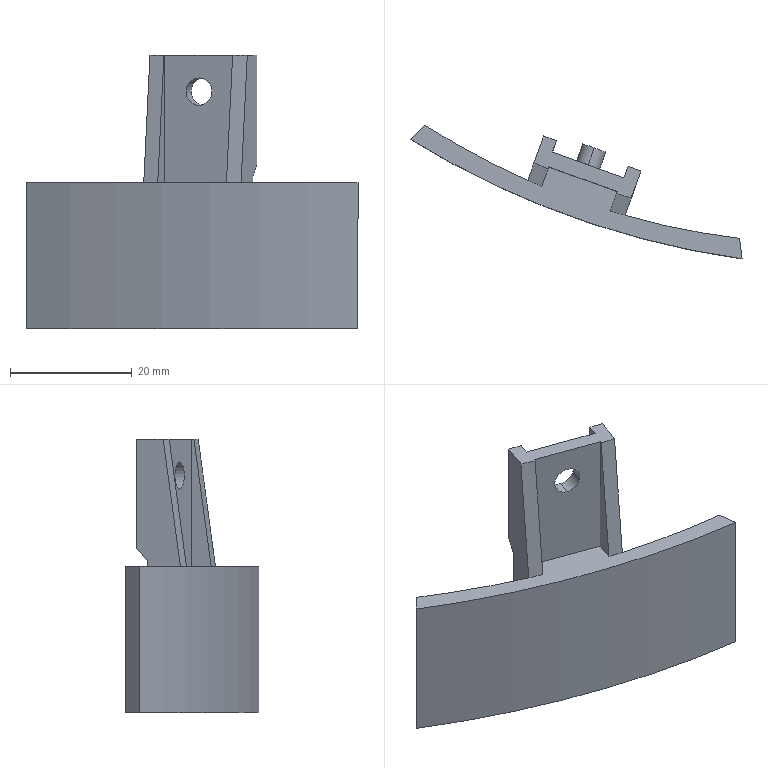Component | SolidWorks | CLS-MechanismIndicatorPlate-1 | 1 solid | 32 faces | box 54.57 x 21.97 x 45 mm | volume 6378 mm3 | plane 23 | cylinder 7 | cone 2 | commonest cylinder face diameters 4 x2 4.5 x2 247.05 x2 283.333 x1
STEP:
#1=CARTESIAN_POINT('',(1.558,-2.417,-0.8662));
#2=VERTEX_POINT('',#1);
#3=CARTESIAN_POINT('',(1.558,-2.417,-0.7087));
#4=VERTEX_POINT('',#3);
#5=CARTESIAN_POINT('',(1.558,-2.417,-0.7874));
#6=DIRECTION('',(0.3389,0.9408,-0.));
#7=DIRECTION('',(0.,-0.,-1.));
#8=AXIS2_PLACEMENT_3D('',#5,#6,#7);
#9=CIRCLE('',#8,0.07874);
#10=EDGE_CURVE('',#2,#4,#9,.T.);
#11=ORIENTED_EDGE('',*,*,#10,.F.);
#12=CARTESIAN_POINT('',(1.518,-2.528,-0.8662));
#13=VERTEX_POINT('',#12);
#14=CARTESIAN_POINT('',(1.558,-2.417,-0.8662));
#15=DIRECTION('',(-0.3389,-0.9408,0.));
#16=VECTOR('',#15,39.37);
#17=LINE('',#14,#16);
#18=EDGE_CURVE('',#2,#13,#17,.T.);
#19=ORIENTED_EDGE('',*,*,#18,.T.);
#20=CARTESIAN_POINT('',(1.518,-2.528,-0.7087));
#21=VERTEX_POINT('',#20);
#22=CARTESIAN_POINT('',(1.518,-2.528,-0.7874));
#23=DIRECTION('',(0.3389,0.9408,-0.));
#24=DIRECTION('',(0.,0.,-1.));
#25=AXIS2_PLACEMENT_3D('',#22,#23,#24);
#26=CIRCLE('',#25,0.07874);
#27=EDGE_CURVE('',#13,#21,#26,.T.);
#28=ORIENTED_EDGE('',*,*,#27,.T.);
#29=CARTESIAN_POINT('',(1.558,-2.417,-0.7087));
#30=DIRECTION('',(-0.3389,-0.9408,0.));
#31=VECTOR('',#30,39.37);
#32=LINE('',#29,#31);
#33=EDGE_CURVE('',#4,#21,#32,.T.);
#34=ORIENTED_EDGE('',*,*,#33,.F.);
#35=EDGE_LOOP('',(#11,#19,#28,#34));
#36=FACE_OUTER_BOUND('',#35,.T.);
#37=CARTESIAN_POINT('',(1.558,-2.417,-0.7874));
#38=DIRECTION('',(-0.3389,-0.9408,0.));
#39=DIRECTION('',(0.,0.,1.));
#40=AXIS2_PLACEMENT_3D('',#37,#38,#39);
#41=CYLINDRICAL_SURFACE('',#40,0.07874);
#42=ADVANCED_FACE('',(#36),#41,.T.);
#43=CARTESIAN_POINT('',(1.485,-2.62,-0.3051));
#44=VERTEX_POINT('',#43);
#45=CARTESIAN_POINT('',(1.485,-2.62,-0.4823));
#46=VERTEX_POINT('',#45);
#47=CARTESIAN_POINT('',(1.485,-2.62,-0.3937));
#48=DIRECTION('',(0.3389,0.9408,-0.));
#49=DIRECTION('',(-0.9408,0.3389,0.));
#50=AXIS2_PLACEMENT_3D('',#47,#48,#49);
#51=CIRCLE('',#50,0.08858);
#52=EDGE_CURVE('',#44,#46,#51,.T.);
#53=ORIENTED_EDGE('',*,*,#52,.F.);
#54=CARTESIAN_POINT('',(1.518,-2.528,-0.3051));
#55=VERTEX_POINT('',#54);
#56=CARTESIAN_POINT('',(1.425,-2.787,-0.3051));
#57=DIRECTION('',(0.3389,0.9408,-0.));
#58=VECTOR('',#57,39.37);
#59=LINE('',#56,#58);
#60=EDGE_CURVE('',#44,#55,#59,.T.);
#61=ORIENTED_EDGE('',*,*,#60,.T.);
#62=CARTESIAN_POINT('',(1.518,-2.528,-0.4823));
#63=VERTEX_POINT('',#62);
#64=CARTESIAN_POINT('',(1.518,-2.528,-0.3937));
#65=DIRECTION('',(0.3389,0.9408,-0.));
#66=DIRECTION('',(0.,-0.,-1.));
#67=AXIS2_PLACEMENT_3D('',#64,#65,#66);
#68=CIRCLE('',#67,0.08858);
#69=EDGE_CURVE('',#55,#63,#68,.T.);
#70=ORIENTED_EDGE('',*,*,#69,.T.);
#71=CARTESIAN_POINT('',(1.425,-2.787,-0.4823));
#72=DIRECTION('',(0.3389,0.9408,-0.));
#73=VECTOR('',#72,39.37);
#74=LINE('',#71,#73);
#75=EDGE_CURVE('',#46,#63,#74,.T.);
#76=ORIENTED_EDGE('',*,*,#75,.F.);
#77=EDGE_LOOP('',(#53,#61,#70,#76));
#78=FACE_OUTER_BOUND('',#77,.T.);
#79=CARTESIAN_POINT('',(1.425,-2.787,-0.3937));
#80=DIRECTION('',(0.3389,0.9408,-0.));
#81=DIRECTION('',(0.,-0.,-1.));
#82=AXIS2_PLACEMENT_3D('',#79,#80,#81);
#83=CYLINDRICAL_SURFACE('',#82,0.08858);
#84=ADVANCED_FACE('',(#78),#83,.F.);
#85=CARTESIAN_POINT('',(1.287,-2.444,-0.9449));
#86=VERTEX_POINT('',#85);
#87=CARTESIAN_POINT('',(1.203,-2.414,-0.9449));
#88=VERTEX_POINT('',#87);
#89=CARTESIAN_POINT('',(1.287,-2.444,-0.9449));
#90=DIRECTION('',(-0.9408,0.3389,0.));
#91=VECTOR('',#90,39.37);
#92=LINE('',#89,#91);
#93=EDGE_CURVE('',#86,#88,#92,.T.);
#94=ORIENTED_EDGE('',*,*,#93,.F.);
#95=CARTESIAN_POINT('',(1.287,-2.444,-0.1575));
#96=VERTEX_POINT('',#95);
#97=CARTESIAN_POINT('',(1.287,-2.444,-0.1575));
#98=DIRECTION('',(-0.,-0.,-1.));
#99=VECTOR('',#98,39.37);
#100=LINE('',#97,#99);
#101=EDGE_CURVE('',#96,#86,#100,.T.);
#102=ORIENTED_EDGE('',*,*,#101,.F.);
#103=CARTESIAN_POINT('',(1.75,-2.611,-0.1575));
#104=VERTEX_POINT('',#103);
#105=CARTESIAN_POINT('',(1.203,-2.414,-0.1575));
#106=DIRECTION('',(-0.9408,0.3389,0.));
#107=VECTOR('',#106,39.37);
#108=LINE('',#105,#107);
#109=EDGE_CURVE('',#104,#96,#108,.T.);
#110=ORIENTED_EDGE('',*,*,#109,.F.);
#111=CARTESIAN_POINT('',(1.75,-2.611,-0.9449));
#112=VERTEX_POINT('',#111);
#113=CARTESIAN_POINT('',(1.75,-2.611,-0.1575));
#114=DIRECTION('',(0.,0.,1.));
#115=VECTOR('',#114,39.37);
#116=LINE('',#113,#115);
#117=EDGE_CURVE('',#112,#104,#116,.T.);
#118=ORIENTED_EDGE('',*,*,#117,.F.);
#119=CARTESIAN_POINT('',(1.833,-2.641,-0.9449));
#120=VERTEX_POINT('',#119);
#121=CARTESIAN_POINT('',(1.833,-2.641,-0.9449));
#122=DIRECTION('',(-0.9408,0.3389,0.));
#123=VECTOR('',#122,39.37);
#124=LINE('',#121,#123);
#125=EDGE_CURVE('',#120,#112,#124,.T.);
#126=ORIENTED_EDGE('',*,*,#125,.F.);
#127=CARTESIAN_POINT('',(1.833,-2.641,-1.929));
#128=VERTEX_POINT('',#127);
#129=CARTESIAN_POINT('',(1.833,-2.641,-0.9843));
#130=DIRECTION('',(-0.,-0.,-1.));
#131=VECTOR('',#130,39.37);
#132=LINE('',#129,#131);
#133=EDGE_CURVE('',#120,#128,#132,.T.);
#134=ORIENTED_EDGE('',*,*,#133,.T.);
#135=CARTESIAN_POINT('',(1.203,-2.414,-1.929));
#136=VERTEX_POINT('',#135);
#137=CARTESIAN_POINT('',(0.4996,-2.161,-1.929));
#138=DIRECTION('',(0.9408,-0.3389,-0.));
#139=VECTOR('',#138,39.37);
#140=LINE('',#137,#139);
#141=EDGE_CURVE('',#136,#128,#140,.T.);
#142=ORIENTED_EDGE('',*,*,#141,.F.);
#143=CARTESIAN_POINT('',(1.203,-2.414,-0.9843));
#144=DIRECTION('',(-0.,-0.,-1.));
#145=VECTOR('',#144,39.37);
#146=LINE('',#143,#145);
#147=EDGE_CURVE('',#88,#136,#146,.T.);
#148=ORIENTED_EDGE('',*,*,#147,.F.);
#149=EDGE_LOOP('',(#94,#102,#110,#118,#126,#134,#142,#148));
#150=FACE_OUTER_BOUND('',#149,.T.);
#151=CARTESIAN_POINT('',(1.314,-2.454,-1.811));
#152=VERTEX_POINT('',#151);
#153=CARTESIAN_POINT('',(1.314,-2.454,-1.095));
#154=VERTEX_POINT('',#153);
#155=CARTESIAN_POINT('',(1.314,-2.454,-1.095));
#156=DIRECTION('',(0.,0.,1.));
#157=VECTOR('',#156,39.37);
#158=LINE('',#155,#157);
#159=EDGE_CURVE('',#152,#154,#158,.T.);
#160=ORIENTED_EDGE('',*,*,#159,.F.);
#161=CARTESIAN_POINT('',(1.722,-2.601,-1.811));
#162=VERTEX_POINT('',#161);
#163=CARTESIAN_POINT('',(1.722,-2.601,-1.811));
#164=DIRECTION('',(-0.9408,0.3389,0.));
#165=VECTOR('',#164,39.37);
#166=LINE('',#163,#165);
#167=EDGE_CURVE('',#162,#152,#166,.T.);
#168=ORIENTED_EDGE('',*,*,#167,.F.);
#169=CARTESIAN_POINT('',(1.722,-2.601,-1.095));
#170=VERTEX_POINT('',#169);
#171=CARTESIAN_POINT('',(1.722,-2.601,-1.095));
#172=DIRECTION('',(-0.,-0.,-1.));
#173=VECTOR('',#172,39.37);
#174=LINE('',#171,#173);
#175=EDGE_CURVE('',#170,#162,#174,.T.);
#176=ORIENTED_EDGE('',*,*,#175,.F.);
#177=CARTESIAN_POINT('',(1.722,-2.601,-1.095));
#178=DIRECTION('',(0.9408,-0.3389,-0.));
#179=VECTOR('',#178,39.37);
#180=LINE('',#177,#179);
#181=EDGE_CURVE('',#154,#170,#180,.T.);
#182=ORIENTED_EDGE('',*,*,#181,.F.);
#183=EDGE_LOOP('',(#160,#168,#176,#182));
#184=FACE_BOUND('',#183,.T.);
#185=CARTESIAN_POINT('',(1.518,-2.528,-0.3937));
#186=DIRECTION('',(0.3389,0.9408,-0.));
#187=DIRECTION('',(0.,-0.,-1.));
#188=AXIS2_PLACEMENT_3D('',#185,#186,#187);
#189=CIRCLE('',#188,0.08858);
#190=EDGE_CURVE('',#63,#55,#189,.T.);
#191=ORIENTED_EDGE('',*,*,#190,.F.);
#192=ORIENTED_EDGE('',*,*,#69,.F.);
#193=EDGE_LOOP('',(#191,#192));
#194=FACE_BOUND('',#193,.T.);
#195=CARTESIAN_POINT('',(1.518,-2.528,-0.7874));
#196=DIRECTION('',(0.3389,0.9408,-0.));
#197=DIRECTION('',(0.,0.,-1.));
#198=AXIS2_PLACEMENT_3D('',#195,#196,#197);
#199=CIRCLE('',#198,0.07874);
#200=EDGE_CURVE('',#21,#13,#199,.T.);
#201=ORIENTED_EDGE('',*,*,#200,.F.);
#202=ORIENTED_EDGE('',*,*,#27,.F.);
#203=EDGE_LOOP('',(#201,#202));
#204=FACE_BOUND('',#203,.T.);
#205=CARTESIAN_POINT('',(0.4996,-2.161,-0.9843));
#206=DIRECTION('',(0.3389,0.9408,-0.));
#207=DIRECTION('',(-0.,-0.,-1.));
#208=AXIS2_PLACEMENT_3D('',#205,#206,#207);
#209=PLANE('',#208);
#210=ADVANCED_FACE('',(#150,#184,#194,#204),#209,.T.);
#211=CARTESIAN_POINT('',(1.258,-2.553,-0.1575));
#212=VERTEX_POINT('',#211);
#213=CARTESIAN_POINT('',(1.218,-2.665,-0.9843));
#214=VERTEX_POINT('',#213);
#215=CARTESIAN_POINT('',(1.258,-2.553,-0.1575));
#216=CARTESIAN_POINT('',(1.246,-2.585,-0.3966));
#217=CARTESIAN_POINT('',(1.235,-2.618,-0.6356));
#218=CARTESIAN_POINT('',(1.223,-2.65,-0.8747));
#219=CARTESIAN_POINT('',(1.221,-2.655,-0.9112));
#220=CARTESIAN_POINT('',(1.22,-2.66,-0.9477));
#221=CARTESIAN_POINT('',(1.218,-2.665,-0.9843));
#222=B_SPLINE_CURVE_WITH_KNOTS('',3,(#215,#216,#217,#218,#219,#220,#221),.UNSPECIFIED.,.F.,.F.,(4,3,4),(0.02067,0.03908,0.04189),.UNSPECIFIED.);
#223=EDGE_CURVE('',#212,#214,#222,.T.);
#224=ORIENTED_EDGE('',*,*,#223,.F.);
#225=CARTESIAN_POINT('',(1.167,-2.514,-0.1575));
#226=VERTEX_POINT('',#225);
#227=CARTESIAN_POINT('',(3.086,1.825,-0.1575));
#228=DIRECTION('',(0.,0.,1.));
#229=DIRECTION('',(0.9408,-0.3389,-0.));
#230=AXIS2_PLACEMENT_3D('',#227,#228,#229);
#231=CIRCLE('',#230,4.745);
#232=EDGE_CURVE('',#226,#212,#231,.T.);
#233=ORIENTED_EDGE('',*,*,#232,.F.);
#234=CARTESIAN_POINT('',(1.127,-2.626,-0.9843));
#235=VERTEX_POINT('',#234);
#236=CARTESIAN_POINT('',(1.127,-2.626,-0.9843));
#237=CARTESIAN_POINT('',(1.141,-2.589,-0.7087));
#238=CARTESIAN_POINT('',(1.154,-2.551,-0.4331));
#239=CARTESIAN_POINT('',(1.167,-2.514,-0.1575));
#240=B_SPLINE_CURVE_WITH_KNOTS('',3,(#236,#237,#238,#239),.UNSPECIFIED.,.F.,.F.,(4,4),(0.,0.02121),.UNSPECIFIED.);
#241=EDGE_CURVE('',#235,#226,#240,.T.);
#242=ORIENTED_EDGE('',*,*,#241,.F.);
#243=CARTESIAN_POINT('',(3.086,1.825,-0.9843));
#244=DIRECTION('',(0.,0.,1.));
#245=DIRECTION('',(0.9408,-0.3389,-0.));
#246=AXIS2_PLACEMENT_3D('',#243,#244,#245);
#247=CIRCLE('',#246,4.863);
#248=EDGE_CURVE('',#235,#214,#247,.T.);
#249=ORIENTED_EDGE('',*,*,#248,.T.);
#250=EDGE_LOOP('',(#224,#233,#242,#249));
#251=FACE_OUTER_BOUND('',#250,.T.);
#252=CARTESIAN_POINT('',(3.086,1.825,-0.1575));
#253=DIRECTION('',(-0.,-0.,-1.));
#254=DIRECTION('',(0.9408,-0.3389,-0.));
#255=AXIS2_PLACEMENT_3D('',#252,#253,#254);
#256=CONICAL_SURFACE('',#255,4.745,0.1419);
#257=ADVANCED_FACE('',(#251),#256,.T.);
#258=CARTESIAN_POINT('',(0.3653,-2.359,-1.929));
#259=VERTEX_POINT('',#258);
#260=CARTESIAN_POINT('',(0.4609,-2.268,-1.929));
#261=VERTEX_POINT('',#260);
#262=CARTESIAN_POINT('',(0.4609,-2.268,-1.929));
#263=DIRECTION('',(0.7239,0.6899,-0.));
#264=VECTOR('',#263,39.37);
#265=LINE('',#262,#264);
#266=EDGE_CURVE('',#259,#261,#265,.T.);
#267=ORIENTED_EDGE('',*,*,#266,.F.);
#268=CARTESIAN_POINT('',(0.3653,-2.359,-0.9843));
#269=VERTEX_POINT('',#268);
#270=CARTESIAN_POINT('',(0.3653,-2.359,-0.9843));
#271=DIRECTION('',(-0.,-0.,-1.));
#272=VECTOR('',#271,39.37);
#273=LINE('',#270,#272);
#274=EDGE_CURVE('',#269,#259,#273,.T.);
#275=ORIENTED_EDGE('',*,*,#274,.F.);
#276=CARTESIAN_POINT('',(0.4609,-2.268,-0.9843));
#277=VERTEX_POINT('',#276);
#278=CARTESIAN_POINT('',(0.4609,-2.268,-0.9843));
#279=DIRECTION('',(0.7239,0.6899,-0.));
#280=VECTOR('',#279,39.37);
#281=LINE('',#278,#280);
#282=EDGE_CURVE('',#269,#277,#281,.T.);
#283=ORIENTED_EDGE('',*,*,#282,.T.);
#284=CARTESIAN_POINT('',(0.4609,-2.268,-0.9843));
#285=DIRECTION('',(-0.,-0.,-1.));
#286=VECTOR('',#285,39.37);
#287=LINE('',#284,#286);
#288=EDGE_CURVE('',#277,#261,#287,.T.);
#289=ORIENTED_EDGE('',*,*,#288,.T.);
#290=EDGE_LOOP('',(#267,#275,#283,#289));
#291=FACE_OUTER_BOUND('',#290,.T.);
#292=CARTESIAN_POINT('',(0.4609,-2.268,-0.9843));
#293=DIRECTION('',(-0.6899,0.7239,-0.));
#294=DIRECTION('',(-0.7239,-0.6899,0.));
#295=AXIS2_PLACEMENT_3D('',#292,#293,#294);
#296=PLANE('',#295);
#297=ADVANCED_FACE('',(#291),#296,.T.);
#298=CARTESIAN_POINT('',(2.514,-3.133,-1.929));
#299=VERTEX_POINT('',#298);
#300=CARTESIAN_POINT('',(3.29,2.39,-1.929));
#301=DIRECTION('',(0.,0.,1.));
#302=DIRECTION('',(-0.9408,0.3389,0.));
#303=AXIS2_PLACEMENT_3D('',#300,#301,#302);
#304=CIRCLE('',#303,5.577);
#305=EDGE_CURVE('',#259,#299,#304,.T.);
#306=ORIENTED_EDGE('',*,*,#305,.T.);
#307=CARTESIAN_POINT('',(2.514,-3.133,-0.9843));
#308=VERTEX_POINT('',#307);
#309=CARTESIAN_POINT('',(2.514,-3.133,-0.9843));
#310=DIRECTION('',(-0.,-0.,-1.));
#311=VECTOR('',#310,39.37);
#312=LINE('',#309,#311);
#313=EDGE_CURVE('',#308,#299,#312,.T.);
#314=ORIENTED_EDGE('',*,*,#313,.F.);
#315=CARTESIAN_POINT('',(3.29,2.39,-0.9843));
#316=DIRECTION('',(0.,0.,1.));
#317=DIRECTION('',(-0.9408,0.3389,0.));
#318=AXIS2_PLACEMENT_3D('',#315,#316,#317);
#319=CIRCLE('',#318,5.577);
#320=EDGE_CURVE('',#269,#308,#319,.T.);
#321=ORIENTED_EDGE('',*,*,#320,.F.);
#322=ORIENTED_EDGE('',*,*,#274,.T.);
#323=EDGE_LOOP('',(#306,#314,#321,#322));
#324=FACE_OUTER_BOUND('',#323,.T.);
#325=CARTESIAN_POINT('',(3.29,2.39,-0.9843));
#326=DIRECTION('',(-0.,-0.,-1.));
#327=DIRECTION('',(0.9408,-0.3389,-0.));
#328=AXIS2_PLACEMENT_3D('',#325,#326,#327);
#329=CYLINDRICAL_SURFACE('',#328,5.577);
#330=ADVANCED_FACE('',(#324),#329,.T.);
#331=CARTESIAN_POINT('',(2.498,-3.002,-1.929));
#332=VERTEX_POINT('',#331);
#333=CARTESIAN_POINT('',(2.384,-2.04,-1.929));
#334=DIRECTION('',(-0.1176,0.9931,-0.));
#335=VECTOR('',#334,39.37);
#336=LINE('',#333,#335);
#337=EDGE_CURVE('',#299,#332,#336,.T.);
#338=ORIENTED_EDGE('',*,*,#337,.T.);
#339=CARTESIAN_POINT('',(2.498,-3.002,-0.9843));
#340=VERTEX_POINT('',#339);
#341=CARTESIAN_POINT('',(2.498,-3.002,-0.9843));
#342=DIRECTION('',(-0.,-0.,-1.));
#343=VECTOR('',#342,39.37);
#344=LINE('',#341,#343);
#345=EDGE_CURVE('',#340,#332,#344,.T.);
#346=ORIENTED_EDGE('',*,*,#345,.F.);
#347=CARTESIAN_POINT('',(2.384,-2.04,-0.9843));
#348=DIRECTION('',(-0.1176,0.9931,-0.));
#349=VECTOR('',#348,39.37);
#350=LINE('',#347,#349);
#351=EDGE_CURVE('',#308,#340,#350,.T.);
#352=ORIENTED_EDGE('',*,*,#351,.F.);
#353=ORIENTED_EDGE('',*,*,#313,.T.);
#354=EDGE_LOOP('',(#338,#346,#352,#353));
#355=FACE_OUTER_BOUND('',#354,.T.);
#356=CARTESIAN_POINT('',(2.384,-2.04,-0.9843));
#357=DIRECTION('',(-0.9931,-0.1176,0.));
#358=DIRECTION('',(0.1176,-0.9931,0.));
#359=AXIS2_PLACEMENT_3D('',#356,#357,#358);
#360=PLANE('',#359);
#361=ADVANCED_FACE('',(#355),#360,.F.);
#362=CARTESIAN_POINT('',(1.757,-2.853,-1.929));
#363=VERTEX_POINT('',#362);
#364=CARTESIAN_POINT('',(3.086,1.825,-1.929));
#365=DIRECTION('',(0.,0.,1.));
#366=DIRECTION('',(-0.9408,0.3389,0.));
#367=AXIS2_PLACEMENT_3D('',#364,#365,#366);
#368=CIRCLE('',#367,4.863);
#369=EDGE_CURVE('',#363,#332,#368,.T.);
#370=ORIENTED_EDGE('',*,*,#369,.F.);
#371=CARTESIAN_POINT('',(1.757,-2.853,-0.9843));
#372=VERTEX_POINT('',#371);
#373=CARTESIAN_POINT('',(1.757,-2.853,-0.9843));
#374=DIRECTION('',(-0.,-0.,-1.));
#375=VECTOR('',#374,39.37);
#376=LINE('',#373,#375);
#377=EDGE_CURVE('',#372,#363,#376,.T.);
#378=ORIENTED_EDGE('',*,*,#377,.F.);
#379=CARTESIAN_POINT('',(3.086,1.825,-0.9843));
#380=DIRECTION('',(0.,0.,1.));
#381=DIRECTION('',(-0.9408,0.3389,0.));
#382=AXIS2_PLACEMENT_3D('',#379,#380,#381);
#383=CIRCLE('',#382,4.863);
#384=EDGE_CURVE('',#372,#340,#383,.T.);
#385=ORIENTED_EDGE('',*,*,#384,.T.);
#386=ORIENTED_EDGE('',*,*,#345,.T.);
#387=EDGE_LOOP('',(#370,#378,#385,#386));
#388=FACE_OUTER_BOUND('',#387,.T.);
#389=CARTESIAN_POINT('',(3.086,1.825,-0.9843));
#390=DIRECTION('',(-0.,-0.,-1.));
#391=DIRECTION('',(0.9408,-0.3389,-0.));
#392=AXIS2_PLACEMENT_3D('',#389,#390,#391);
#393=CYLINDRICAL_SURFACE('',#392,4.863);
#394=ADVANCED_FACE('',(#388),#393,.F.);
#395=CARTESIAN_POINT('',(1.797,-2.741,-0.1575));
#396=VERTEX_POINT('',#395);
#397=CARTESIAN_POINT('',(1.86,-2.567,-0.1575));
#398=VERTEX_POINT('',#397);
#399=CARTESIAN_POINT('',(1.833,-2.641,-0.1575));
#400=DIRECTION('',(0.3389,0.9408,-0.));
#401=VECTOR('',#400,39.37);
#402=LINE('',#399,#401);
#403=EDGE_CURVE('',#396,#398,#402,.T.);
#404=ORIENTED_EDGE('',*,*,#403,.F.);
#405=CARTESIAN_POINT('',(1.797,-2.741,-0.1575));
#406=CARTESIAN_POINT('',(1.784,-2.778,-0.4331));
#407=CARTESIAN_POINT('',(1.77,-2.815,-0.7087));
#408=CARTESIAN_POINT('',(1.757,-2.853,-0.9843));
#409=B_SPLINE_CURVE_WITH_KNOTS('',3,(#405,#406,#407,#408),.UNSPECIFIED.,.F.,.F.,(4,4),(0.,0.02121),.UNSPECIFIED.);
#410=EDGE_CURVE('',#396,#372,#409,.T.);
#411=ORIENTED_EDGE('',*,*,#410,.T.);
#412=ORIENTED_EDGE('',*,*,#377,.T.);
#413=CARTESIAN_POINT('',(1.794,-2.749,-1.929));
#414=DIRECTION('',(0.3389,0.9408,-0.));
#415=VECTOR('',#414,39.37);
#416=LINE('',#413,#415);
#417=EDGE_CURVE('',#363,#128,#416,.T.);
#418=ORIENTED_EDGE('',*,*,#417,.T.);
#419=ORIENTED_EDGE('',*,*,#133,.F.);
#420=CARTESIAN_POINT('',(1.86,-2.567,-0.8662));
#421=VERTEX_POINT('',#420);
#422=CARTESIAN_POINT('',(1.86,-2.567,-0.8662));
#423=DIRECTION('',(0.2396,0.6653,0.7071));
#424=VECTOR('',#423,39.37);
#425=LINE('',#422,#424);
#426=EDGE_CURVE('',#120,#421,#425,.T.);
#427=ORIENTED_EDGE('',*,*,#426,.T.);
#428=CARTESIAN_POINT('',(1.86,-2.567,-0.1575));
#429=DIRECTION('',(-0.,-0.,-1.));
#430=VECTOR('',#429,39.37);
#431=LINE('',#428,#430);
#432=EDGE_CURVE('',#398,#421,#431,.T.);
#433=ORIENTED_EDGE('',*,*,#432,.F.);
#434=EDGE_LOOP('',(#404,#411,#412,#418,#419,#427,#433));
#435=FACE_OUTER_BOUND('',#434,.T.);
#436=CARTESIAN_POINT('',(1.794,-2.749,-0.9843));
#437=DIRECTION('',(-0.9408,0.3389,0.));
#438=DIRECTION('',(-0.,-0.,-1.));
#439=AXIS2_PLACEMENT_3D('',#436,#437,#438);
#440=PLANE('',#439);
#441=ADVANCED_FACE('',(#435),#440,.F.);
#442=CARTESIAN_POINT('',(1.127,-2.626,-1.929));
#443=VERTEX_POINT('',#442);
#444=CARTESIAN_POINT('',(1.127,-2.626,-0.9843));
#445=DIRECTION('',(-0.,-0.,-1.));
#446=VECTOR('',#445,39.37);
#447=LINE('',#444,#446);
#448=EDGE_CURVE('',#235,#443,#447,.T.);
#449=ORIENTED_EDGE('',*,*,#448,.F.);
#450=ORIENTED_EDGE('',*,*,#241,.T.);
#451=CARTESIAN_POINT('',(1.23,-2.34,-0.1575));
#452=VERTEX_POINT('',#451);
#453=CARTESIAN_POINT('',(1.203,-2.414,-0.1575));
#454=DIRECTION('',(-0.3389,-0.9408,0.));
#455=VECTOR('',#454,39.37);
#456=LINE('',#453,#455);
#457=EDGE_CURVE('',#452,#226,#456,.T.);
#458=ORIENTED_EDGE('',*,*,#457,.F.);
#459=CARTESIAN_POINT('',(1.23,-2.34,-0.8662));
#460=VERTEX_POINT('',#459);
#461=CARTESIAN_POINT('',(1.23,-2.34,-0.1575));
#462=DIRECTION('',(0.,0.,1.));
#463=VECTOR('',#462,39.37);
#464=LINE('',#461,#463);
#465=EDGE_CURVE('',#460,#452,#464,.T.);
#466=ORIENTED_EDGE('',*,*,#465,.F.);
#467=CARTESIAN_POINT('',(1.177,-2.487,-1.022));
#468=DIRECTION('',(-0.2396,-0.6653,-0.7071));
#469=VECTOR('',#468,39.37);
#470=LINE('',#467,#469);
#471=EDGE_CURVE('',#460,#88,#470,.T.);
#472=ORIENTED_EDGE('',*,*,#471,.T.);
#473=ORIENTED_EDGE('',*,*,#147,.T.);
#474=CARTESIAN_POINT('',(1.165,-2.522,-1.929));
#475=DIRECTION('',(0.3389,0.9408,-0.));
#476=VECTOR('',#475,39.37);
#477=LINE('',#474,#476);
#478=EDGE_CURVE('',#443,#136,#477,.T.);
#479=ORIENTED_EDGE('',*,*,#478,.F.);
#480=EDGE_LOOP('',(#449,#450,#458,#466,#472,#473,#479));
#481=FACE_OUTER_BOUND('',#480,.T.);
#482=CARTESIAN_POINT('',(1.165,-2.522,-0.9843));
#483=DIRECTION('',(-0.9408,0.3389,0.));
#484=DIRECTION('',(-0.,-0.,-1.));
#485=AXIS2_PLACEMENT_3D('',#482,#483,#484);
#486=PLANE('',#485);
#487=ADVANCED_FACE('',(#481),#486,.T.);
#488=CARTESIAN_POINT('',(3.086,1.825,-1.929));
#489=DIRECTION('',(0.,0.,1.));
#490=DIRECTION('',(-0.9408,0.3389,0.));
#491=AXIS2_PLACEMENT_3D('',#488,#489,#490);
#492=CIRCLE('',#491,4.863);
#493=EDGE_CURVE('',#261,#443,#492,.T.);
#494=ORIENTED_EDGE('',*,*,#493,.F.);
#495=ORIENTED_EDGE('',*,*,#288,.F.);
#496=CARTESIAN_POINT('',(3.086,1.825,-0.9843));
#497=DIRECTION('',(0.,0.,1.));
#498=DIRECTION('',(-0.9408,0.3389,0.));
#499=AXIS2_PLACEMENT_3D('',#496,#497,#498);
#500=CIRCLE('',#499,4.863);
#501=EDGE_CURVE('',#277,#235,#500,.T.);
#502=ORIENTED_EDGE('',*,*,#501,.T.);
#503=ORIENTED_EDGE('',*,*,#448,.T.);
#504=EDGE_LOOP('',(#494,#495,#502,#503));
#505=FACE_OUTER_BOUND('',#504,.T.);
#506=CARTESIAN_POINT('',(3.086,1.825,-0.9843));
#507=DIRECTION('',(-0.,-0.,-1.));
#508=DIRECTION('',(0.9408,-0.3389,-0.));
#509=AXIS2_PLACEMENT_3D('',#506,#507,#508);
#510=CYLINDRICAL_SURFACE('',#509,4.863);
#511=ADVANCED_FACE('',(#505),#510,.F.);
#512=CARTESIAN_POINT('',(1.662,-2.825,-0.9843));
#513=VERTEX_POINT('',#512);
#514=CARTESIAN_POINT('',(3.086,1.825,-0.9843));
#515=DIRECTION('',(0.,0.,1.));
#516=DIRECTION('',(0.9408,-0.3389,-0.));
#517=AXIS2_PLACEMENT_3D('',#514,#515,#516);
#518=CIRCLE('',#517,4.863);
#519=EDGE_CURVE('',#513,#372,#518,.T.);
#520=ORIENTED_EDGE('',*,*,#519,.F.);
#521=CARTESIAN_POINT('',(1.707,-2.7,-0.9843));
#522=VERTEX_POINT('',#521);
#523=CARTESIAN_POINT('',(1.707,-2.7,-0.9843));
#524=DIRECTION('',(0.3389,0.9408,-0.));
#525=VECTOR('',#524,39.37);
#526=LINE('',#523,#525);
#527=EDGE_CURVE('',#513,#522,#526,.T.);
#528=ORIENTED_EDGE('',*,*,#527,.T.);
#529=CARTESIAN_POINT('',(1.263,-2.54,-0.9843));
#530=VERTEX_POINT('',#529);
#531=CARTESIAN_POINT('',(1.263,-2.54,-0.9843));
#532=DIRECTION('',(-0.9408,0.3389,0.));
#533=VECTOR('',#532,39.37);
#534=LINE('',#531,#533);
#535=EDGE_CURVE('',#522,#530,#534,.T.);
#536=ORIENTED_EDGE('',*,*,#535,.T.);
#537=CARTESIAN_POINT('',(1.263,-2.54,-0.9843));
#538=DIRECTION('',(-0.3389,-0.9408,0.));
#539=VECTOR('',#538,39.37);
#540=LINE('',#537,#539);
#541=EDGE_CURVE('',#530,#214,#540,.T.);
#542=ORIENTED_EDGE('',*,*,#541,.T.);
#543=ORIENTED_EDGE('',*,*,#248,.F.);
#544=ORIENTED_EDGE('',*,*,#501,.F.);
#545=ORIENTED_EDGE('',*,*,#282,.F.);
#546=ORIENTED_EDGE('',*,*,#320,.T.);
#547=ORIENTED_EDGE('',*,*,#351,.T.);
#548=ORIENTED_EDGE('',*,*,#384,.F.);
#549=EDGE_LOOP('',(#520,#528,#536,#542,#543,#544,#545,#546,#547,#548));
#550=FACE_OUTER_BOUND('',#549,.T.);
#551=CARTESIAN_POINT('',(0.4609,-2.268,-0.9843));
#552=DIRECTION('',(0.,0.,1.));
#553=DIRECTION('',(-0.9408,0.3389,0.));
#554=AXIS2_PLACEMENT_3D('',#551,#552,#553);
#555=PLANE('',#554);
#556=ADVANCED_FACE('',(#550),#555,.T.);
#557=ORIENTED_EDGE('',*,*,#266,.T.);
#558=ORIENTED_EDGE('',*,*,#493,.T.);
#559=ORIENTED_EDGE('',*,*,#478,.T.);
#560=ORIENTED_EDGE('',*,*,#141,.T.);
#561=ORIENTED_EDGE('',*,*,#417,.F.);
#562=ORIENTED_EDGE('',*,*,#369,.T.);
#563=ORIENTED_EDGE('',*,*,#337,.F.);
#564=ORIENTED_EDGE('',*,*,#305,.F.);
#565=EDGE_LOOP('',(#557,#558,#559,#560,#561,#562,#563,#564));
#566=FACE_OUTER_BOUND('',#565,.T.);
#567=CARTESIAN_POINT('',(0.4609,-2.268,-1.929));
#568=DIRECTION('',(0.,0.,1.));
#569=DIRECTION('',(-0.9408,0.3389,0.));
#570=AXIS2_PLACEMENT_3D('',#567,#568,#569);
#571=PLANE('',#570);
#572=ADVANCED_FACE('',(#566),#571,.F.);
#573=ORIENTED_EDGE('',*,*,#232,.T.);
#574=CARTESIAN_POINT('',(1.263,-2.54,-0.1575));
#575=VERTEX_POINT('',#574);
#576=CARTESIAN_POINT('',(1.263,-2.54,-0.1575));
#577=DIRECTION('',(-0.3389,-0.9408,0.));
#578=VECTOR('',#577,39.37);
#579=LINE('',#576,#578);
#580=EDGE_CURVE('',#575,#212,#579,.T.);
#581=ORIENTED_EDGE('',*,*,#580,.F.);
#582=CARTESIAN_POINT('',(1.707,-2.7,-0.1575));
#583=VERTEX_POINT('',#582);
#584=CARTESIAN_POINT('',(1.263,-2.54,-0.1575));
#585=DIRECTION('',(-0.9408,0.3389,0.));
#586=VECTOR('',#585,39.37);
#587=LINE('',#584,#586);
#588=EDGE_CURVE('',#583,#575,#587,.T.);
#589=ORIENTED_EDGE('',*,*,#588,.F.);
#590=CARTESIAN_POINT('',(1.702,-2.713,-0.1575));
#591=VERTEX_POINT('',#590);
#592=CARTESIAN_POINT('',(1.707,-2.7,-0.1575));
#593=DIRECTION('',(0.3389,0.9408,-0.));
#594=VECTOR('',#593,39.37);
#595=LINE('',#592,#594);
#596=EDGE_CURVE('',#591,#583,#595,.T.);
#597=ORIENTED_EDGE('',*,*,#596,.F.);
#598=CARTESIAN_POINT('',(3.086,1.825,-0.1575));
#599=DIRECTION('',(0.,0.,1.));
#600=DIRECTION('',(0.9408,-0.3389,-0.));
#601=AXIS2_PLACEMENT_3D('',#598,#599,#600);
#602=CIRCLE('',#601,4.745);
#603=EDGE_CURVE('',#591,#396,#602,.T.);
#604=ORIENTED_EDGE('',*,*,#603,.T.);
#605=ORIENTED_EDGE('',*,*,#403,.T.);
#606=CARTESIAN_POINT('',(1.776,-2.537,-0.1575));
#607=VERTEX_POINT('',#606);
#608=CARTESIAN_POINT('',(1.86,-2.567,-0.1575));
#609=DIRECTION('',(0.9408,-0.3389,-0.));
#610=VECTOR('',#609,39.37);
#611=LINE('',#608,#610);
#612=EDGE_CURVE('',#607,#398,#611,.T.);
#613=ORIENTED_EDGE('',*,*,#612,.F.);
#614=CARTESIAN_POINT('',(1.776,-2.537,-0.1575));
#615=DIRECTION('',(-0.3389,-0.9408,0.));
#616=VECTOR('',#615,39.37);
#617=LINE('',#614,#616);
#618=EDGE_CURVE('',#607,#104,#617,.T.);
#619=ORIENTED_EDGE('',*,*,#618,.T.);
#620=ORIENTED_EDGE('',*,*,#109,.T.);
#621=CARTESIAN_POINT('',(1.313,-2.37,-0.1575));
#622=VERTEX_POINT('',#621);
#623=CARTESIAN_POINT('',(1.313,-2.37,-0.1575));
#624=DIRECTION('',(-0.3389,-0.9408,0.));
#625=VECTOR('',#624,39.37);
#626=LINE('',#623,#625);
#627=EDGE_CURVE('',#622,#96,#626,.T.);
#628=ORIENTED_EDGE('',*,*,#627,.F.);
#629=CARTESIAN_POINT('',(1.313,-2.37,-0.1575));
#630=DIRECTION('',(0.9408,-0.3389,-0.));
#631=VECTOR('',#630,39.37);
#632=LINE('',#629,#631);
#633=EDGE_CURVE('',#452,#622,#632,.T.);
#634=ORIENTED_EDGE('',*,*,#633,.F.);
#635=ORIENTED_EDGE('',*,*,#457,.T.);
#636=EDGE_LOOP('',(#573,#581,#589,#597,#604,#605,#613,#619,#620,#628,#634,#635));
#637=FACE_OUTER_BOUND('',#636,.T.);
#638=CARTESIAN_POINT('',(3.086,1.825,-0.1575));
#639=DIRECTION('',(-0.,-0.,-1.));
#640=DIRECTION('',(0.9408,-0.3389,-0.));
#641=AXIS2_PLACEMENT_3D('',#638,#639,#640);
#642=PLANE('',#641);
#643=ADVANCED_FACE('',(#637),#642,.F.);
#644=CARTESIAN_POINT('',(1.776,-2.537,-0.8662));
#645=VERTEX_POINT('',#644);
#646=CARTESIAN_POINT('',(1.776,-2.537,-0.1575));
#647=DIRECTION('',(0.,0.,1.));
#648=VECTOR('',#647,39.37);
#649=LINE('',#646,#648);
#650=EDGE_CURVE('',#645,#607,#649,.T.);
#651=ORIENTED_EDGE('',*,*,#650,.F.);
#652=CARTESIAN_POINT('',(1.776,-2.537,-0.8662));
#653=DIRECTION('',(-0.2396,-0.6653,-0.7071));
#654=VECTOR('',#653,39.37);
#655=LINE('',#652,#654);
#656=EDGE_CURVE('',#645,#112,#655,.T.);
#657=ORIENTED_EDGE('',*,*,#656,.T.);
#658=ORIENTED_EDGE('',*,*,#117,.T.);
#659=ORIENTED_EDGE('',*,*,#618,.F.);
#660=EDGE_LOOP('',(#651,#657,#658,#659));
#661=FACE_OUTER_BOUND('',#660,.T.);
#662=CARTESIAN_POINT('',(1.776,-2.537,-0.1575));
#663=DIRECTION('',(0.9408,-0.3389,-0.));
#664=DIRECTION('',(0.,0.,1.));
#665=AXIS2_PLACEMENT_3D('',#662,#663,#664);
#666=PLANE('',#665);
#667=ADVANCED_FACE('',(#661),#666,.F.);
#668=ORIENTED_EDGE('',*,*,#432,.T.);
#669=CARTESIAN_POINT('',(1.776,-2.537,-0.8662));
#670=DIRECTION('',(-0.9408,0.3389,0.));
#671=VECTOR('',#670,39.37);
#672=LINE('',#669,#671);
#673=EDGE_CURVE('',#421,#645,#672,.T.);
#674=ORIENTED_EDGE('',*,*,#673,.T.);
#675=ORIENTED_EDGE('',*,*,#650,.T.);
#676=ORIENTED_EDGE('',*,*,#612,.T.);
#677=EDGE_LOOP('',(#668,#674,#675,#676));
#678=FACE_OUTER_BOUND('',#677,.T.);
#679=CARTESIAN_POINT('',(1.776,-2.537,-0.1575));
#680=DIRECTION('',(-0.3389,-0.9408,0.));
#681=DIRECTION('',(0.,0.,1.));
#682=AXIS2_PLACEMENT_3D('',#679,#680,#681);
#683=PLANE('',#682);
#684=ADVANCED_FACE('',(#678),#683,.F.);
#685=ORIENTED_EDGE('',*,*,#101,.T.);
#686=CARTESIAN_POINT('',(1.313,-2.37,-0.8662));
#687=VERTEX_POINT('',#686);
#688=CARTESIAN_POINT('',(1.313,-2.37,-0.8662));
#689=DIRECTION('',(0.2396,0.6653,0.7071));
#690=VECTOR('',#689,39.37);
#691=LINE('',#688,#690);
#692=EDGE_CURVE('',#86,#687,#691,.T.);
#693=ORIENTED_EDGE('',*,*,#692,.T.);
#694=CARTESIAN_POINT('',(1.313,-2.37,-0.1575));
#695=DIRECTION('',(-0.,-0.,-1.));
#696=VECTOR('',#695,39.37);
#697=LINE('',#694,#696);
#698=EDGE_CURVE('',#622,#687,#697,.T.);
#699=ORIENTED_EDGE('',*,*,#698,.F.);
#700=ORIENTED_EDGE('',*,*,#627,.T.);
#701=EDGE_LOOP('',(#685,#693,#699,#700));
#702=FACE_OUTER_BOUND('',#701,.T.);
#703=CARTESIAN_POINT('',(1.313,-2.37,-0.1575));
#704=DIRECTION('',(-0.9408,0.3389,0.));
#705=DIRECTION('',(-0.,-0.,-1.));
#706=AXIS2_PLACEMENT_3D('',#703,#704,#705);
#707=PLANE('',#706);
#708=ADVANCED_FACE('',(#702),#707,.F.);
#709=ORIENTED_EDGE('',*,*,#698,.T.);
#710=CARTESIAN_POINT('',(1.23,-2.34,-0.8662));
#711=DIRECTION('',(-0.9408,0.3389,0.));
#712=VECTOR('',#711,39.37);
#713=LINE('',#710,#712);
#714=EDGE_CURVE('',#687,#460,#713,.T.);
#715=ORIENTED_EDGE('',*,*,#714,.T.);
#716=ORIENTED_EDGE('',*,*,#465,.T.);
#717=ORIENTED_EDGE('',*,*,#633,.T.);
#718=EDGE_LOOP('',(#709,#715,#716,#717));
#719=FACE_OUTER_BOUND('',#718,.T.);
#720=CARTESIAN_POINT('',(1.313,-2.37,-0.9449));
#721=DIRECTION('',(0.3389,0.9408,-0.));
#722=DIRECTION('',(-0.,-0.,-1.));
#723=AXIS2_PLACEMENT_3D('',#720,#721,#722);
#724=PLANE('',#723);
#725=ADVANCED_FACE('',(#719),#724,.T.);
#726=ORIENTED_EDGE('',*,*,#426,.F.);
#727=ORIENTED_EDGE('',*,*,#125,.T.);
#728=ORIENTED_EDGE('',*,*,#656,.F.);
#729=ORIENTED_EDGE('',*,*,#673,.F.);
#730=EDGE_LOOP('',(#726,#727,#728,#729));
#731=FACE_OUTER_BOUND('',#730,.T.);
#732=CARTESIAN_POINT('',(1.776,-2.537,-0.8662));
#733=DIRECTION('',(-0.2396,-0.6653,0.7071));
#734=DIRECTION('',(0.2396,0.6653,0.7071));
#735=AXIS2_PLACEMENT_3D('',#732,#733,#734);
#736=PLANE('',#735);
#737=ADVANCED_FACE('',(#731),#736,.F.);
#738=ORIENTED_EDGE('',*,*,#692,.F.);
#739=ORIENTED_EDGE('',*,*,#93,.T.);
#740=ORIENTED_EDGE('',*,*,#471,.F.);
#741=ORIENTED_EDGE('',*,*,#714,.F.);
#742=EDGE_LOOP('',(#738,#739,#740,#741));
#743=FACE_OUTER_BOUND('',#742,.T.);
#744=CARTESIAN_POINT('',(1.313,-2.37,-0.8662));
#745=DIRECTION('',(0.2396,0.6653,-0.7071));
#746=DIRECTION('',(-0.2396,-0.6653,-0.7071));
#747=AXIS2_PLACEMENT_3D('',#744,#745,#746);
#748=PLANE('',#747);
#749=ADVANCED_FACE('',(#743),#748,.T.);
#750=CARTESIAN_POINT('',(1.662,-2.825,-0.9843));
#751=CARTESIAN_POINT('',(1.664,-2.82,-0.9477));
#752=CARTESIAN_POINT('',(1.666,-2.815,-0.9112));
#753=CARTESIAN_POINT('',(1.668,-2.81,-0.8747));
#754=CARTESIAN_POINT('',(1.679,-2.778,-0.6356));
#755=CARTESIAN_POINT('',(1.691,-2.746,-0.3966));
#756=CARTESIAN_POINT('',(1.702,-2.713,-0.1575));
#757=B_SPLINE_CURVE_WITH_KNOTS('',3,(#750,#751,#752,#753,#754,#755,#756),.UNSPECIFIED.,.F.,.F.,(4,3,4),(0.03626,0.03908,0.05748),.UNSPECIFIED.);
#758=EDGE_CURVE('',#513,#591,#757,.T.);
#759=ORIENTED_EDGE('',*,*,#758,.F.);
#760=ORIENTED_EDGE('',*,*,#519,.T.);
#761=ORIENTED_EDGE('',*,*,#410,.F.);
#762=ORIENTED_EDGE('',*,*,#603,.F.);
#763=EDGE_LOOP('',(#759,#760,#761,#762));
#764=FACE_OUTER_BOUND('',#763,.T.);
#765=CARTESIAN_POINT('',(3.086,1.825,-0.1575));
#766=DIRECTION('',(-0.,-0.,-1.));
#767=DIRECTION('',(0.9408,-0.3389,-0.));
#768=AXIS2_PLACEMENT_3D('',#765,#766,#767);
#769=CONICAL_SURFACE('',#768,4.745,0.1419);
#770=ADVANCED_FACE('',(#764),#769,.T.);
#771=ORIENTED_EDGE('',*,*,#223,.T.);
#772=ORIENTED_EDGE('',*,*,#541,.F.);
#773=CARTESIAN_POINT('',(1.263,-2.54,-0.9843));
#774=DIRECTION('',(0.,0.,1.));
#775=VECTOR('',#774,39.37);
#776=LINE('',#773,#775);
#777=EDGE_CURVE('',#530,#575,#776,.T.);
#778=ORIENTED_EDGE('',*,*,#777,.T.);
#779=ORIENTED_EDGE('',*,*,#580,.T.);
#780=EDGE_LOOP('',(#771,#772,#778,#779));
#781=FACE_OUTER_BOUND('',#780,.T.);
#782=CARTESIAN_POINT('',(1.263,-2.54,-0.9843));
#783=DIRECTION('',(-0.9408,0.3389,0.));
#784=DIRECTION('',(-0.,-0.,-1.));
#785=AXIS2_PLACEMENT_3D('',#782,#783,#784);
#786=PLANE('',#785);
#787=ADVANCED_FACE('',(#781),#786,.F.);
#788=CARTESIAN_POINT('',(1.485,-2.62,-0.3937));
#789=DIRECTION('',(0.3389,0.9408,-0.));
#790=DIRECTION('',(-0.9408,0.3389,0.));
#791=AXIS2_PLACEMENT_3D('',#788,#789,#790);
#792=CIRCLE('',#791,0.08858);
#793=EDGE_CURVE('',#46,#44,#792,.T.);
#794=ORIENTED_EDGE('',*,*,#793,.T.);
#795=ORIENTED_EDGE('',*,*,#52,.T.);
#796=EDGE_LOOP('',(#794,#795));
#797=FACE_BOUND('',#796,.T.);
#798=ORIENTED_EDGE('',*,*,#588,.T.);
#799=ORIENTED_EDGE('',*,*,#777,.F.);
#800=ORIENTED_EDGE('',*,*,#535,.F.);
#801=CARTESIAN_POINT('',(1.707,-2.7,-0.9843));
#802=DIRECTION('',(0.,0.,1.));
#803=VECTOR('',#802,39.37);
#804=LINE('',#801,#803);
#805=EDGE_CURVE('',#522,#583,#804,.T.);
#806=ORIENTED_EDGE('',*,*,#805,.T.);
#807=EDGE_LOOP('',(#798,#799,#800,#806));
#808=FACE_OUTER_BOUND('',#807,.T.);
#809=CARTESIAN_POINT('',(1.263,-2.54,-0.9843));
#810=DIRECTION('',(0.3389,0.9408,-0.));
#811=DIRECTION('',(-0.9408,0.3389,0.));
#812=AXIS2_PLACEMENT_3D('',#809,#810,#811);
#813=PLANE('',#812);
#814=ADVANCED_FACE('',(#797,#808),#813,.F.);
#815=ORIENTED_EDGE('',*,*,#758,.T.);
#816=ORIENTED_EDGE('',*,*,#596,.T.);
#817=ORIENTED_EDGE('',*,*,#805,.F.);
#818=ORIENTED_EDGE('',*,*,#527,.F.);
#819=EDGE_LOOP('',(#815,#816,#817,#818));
#820=FACE_OUTER_BOUND('',#819,.T.);
#821=CARTESIAN_POINT('',(1.707,-2.7,-0.9843));
#822=DIRECTION('',(0.9408,-0.3389,-0.));
#823=DIRECTION('',(0.,0.,1.));
#824=AXIS2_PLACEMENT_3D('',#821,#822,#823);
#825=PLANE('',#824);
#826=ADVANCED_FACE('',(#820),#825,.F.);
#827=ORIENTED_EDGE('',*,*,#159,.T.);
#828=CARTESIAN_POINT('',(1.221,-2.714,-1.095));
#829=VERTEX_POINT('',#828);
#830=CARTESIAN_POINT('',(1.221,-2.714,-1.095));
#831=DIRECTION('',(0.3389,0.9408,-0.));
#832=VECTOR('',#831,39.37);
#833=LINE('',#830,#832);
#834=EDGE_CURVE('',#829,#154,#833,.T.);
#835=ORIENTED_EDGE('',*,*,#834,.F.);
#836=CARTESIAN_POINT('',(1.221,-2.714,-1.811));
#837=VERTEX_POINT('',#836);
#838=CARTESIAN_POINT('',(1.221,-2.714,-1.095));
#839=DIRECTION('',(0.,0.,1.));
#840=VECTOR('',#839,39.37);
#841=LINE('',#838,#840);
#842=EDGE_CURVE('',#837,#829,#841,.T.);
#843=ORIENTED_EDGE('',*,*,#842,.F.);
#844=CARTESIAN_POINT('',(1.221,-2.714,-1.811));
#845=DIRECTION('',(0.3389,0.9408,-0.));
#846=VECTOR('',#845,39.37);
#847=LINE('',#844,#846);
#848=EDGE_CURVE('',#837,#152,#847,.T.);
#849=ORIENTED_EDGE('',*,*,#848,.T.);
#850=EDGE_LOOP('',(#827,#835,#843,#849));
#851=FACE_OUTER_BOUND('',#850,.T.);
#852=CARTESIAN_POINT('',(1.221,-2.714,-1.095));
#853=DIRECTION('',(-0.9408,0.3389,0.));
#854=DIRECTION('',(-0.,-0.,-1.));
#855=AXIS2_PLACEMENT_3D('',#852,#853,#854);
#856=PLANE('',#855);
#857=ADVANCED_FACE('',(#851),#856,.F.);
#858=ORIENTED_EDGE('',*,*,#167,.T.);
#859=ORIENTED_EDGE('',*,*,#848,.F.);
#860=CARTESIAN_POINT('',(1.629,-2.86,-1.811));
#861=VERTEX_POINT('',#860);
#862=CARTESIAN_POINT('',(1.629,-2.86,-1.811));
#863=DIRECTION('',(-0.9408,0.3389,0.));
#864=VECTOR('',#863,39.37);
#865=LINE('',#862,#864);
#866=EDGE_CURVE('',#861,#837,#865,.T.);
#867=ORIENTED_EDGE('',*,*,#866,.F.);
#868=CARTESIAN_POINT('',(1.629,-2.86,-1.811));
#869=DIRECTION('',(0.3389,0.9408,-0.));
#870=VECTOR('',#869,39.37);
#871=LINE('',#868,#870);
#872=EDGE_CURVE('',#861,#162,#871,.T.);
#873=ORIENTED_EDGE('',*,*,#872,.T.);
#874=EDGE_LOOP('',(#858,#859,#867,#873));
#875=FACE_OUTER_BOUND('',#874,.T.);
#876=CARTESIAN_POINT('',(1.629,-2.86,-1.811));
#877=DIRECTION('',(-0.,-0.,-1.));
#878=DIRECTION('',(0.9408,-0.3389,-0.));
#879=AXIS2_PLACEMENT_3D('',#876,#877,#878);
#880=PLANE('',#879);
#881=ADVANCED_FACE('',(#875),#880,.F.);
#882=ORIENTED_EDGE('',*,*,#175,.T.);
#883=ORIENTED_EDGE('',*,*,#872,.F.);
#884=CARTESIAN_POINT('',(1.629,-2.86,-1.095));
#885=VERTEX_POINT('',#884);
#886=CARTESIAN_POINT('',(1.629,-2.86,-1.095));
#887=DIRECTION('',(-0.,-0.,-1.));
#888=VECTOR('',#887,39.37);
#889=LINE('',#886,#888);
#890=EDGE_CURVE('',#885,#861,#889,.T.);
#891=ORIENTED_EDGE('',*,*,#890,.F.);
#892=CARTESIAN_POINT('',(1.629,-2.86,-1.095));
#893=DIRECTION('',(0.3389,0.9408,-0.));
#894=VECTOR('',#893,39.37);
#895=LINE('',#892,#894);
#896=EDGE_CURVE('',#885,#170,#895,.T.);
#897=ORIENTED_EDGE('',*,*,#896,.T.);
#898=EDGE_LOOP('',(#882,#883,#891,#897));
#899=FACE_OUTER_BOUND('',#898,.T.);
#900=CARTESIAN_POINT('',(1.629,-2.86,-1.095));
#901=DIRECTION('',(0.9408,-0.3389,-0.));
#902=DIRECTION('',(0.,0.,1.));
#903=AXIS2_PLACEMENT_3D('',#900,#901,#902);
#904=PLANE('',#903);
#905=ADVANCED_FACE('',(#899),#904,.F.);
#906=ORIENTED_EDGE('',*,*,#181,.T.);
#907=ORIENTED_EDGE('',*,*,#896,.F.);
#908=CARTESIAN_POINT('',(1.629,-2.86,-1.095));
#909=DIRECTION('',(0.9408,-0.3389,-0.));
#910=VECTOR('',#909,39.37);
#911=LINE('',#908,#910);
#912=EDGE_CURVE('',#829,#885,#911,.T.);
#913=ORIENTED_EDGE('',*,*,#912,.F.);
#914=ORIENTED_EDGE('',*,*,#834,.T.);
#915=EDGE_LOOP('',(#906,#907,#913,#914));
#916=FACE_OUTER_BOUND('',#915,.T.);
#917=CARTESIAN_POINT('',(1.629,-2.86,-1.095));
#918=DIRECTION('',(0.,0.,1.));
#919=DIRECTION('',(-0.9408,0.3389,0.));
#920=AXIS2_PLACEMENT_3D('',#917,#918,#919);
#921=PLANE('',#920);
#922=ADVANCED_FACE('',(#916),#921,.F.);
#923=ORIENTED_EDGE('',*,*,#842,.T.);
#924=ORIENTED_EDGE('',*,*,#912,.T.);
#925=ORIENTED_EDGE('',*,*,#890,.T.);
#926=ORIENTED_EDGE('',*,*,#866,.T.);
#927=EDGE_LOOP('',(#923,#924,#925,#926));
#928=FACE_OUTER_BOUND('',#927,.T.);
#929=CARTESIAN_POINT('',(1.221,-2.714,-1.811));
#930=DIRECTION('',(0.3389,0.9408,-0.));
#931=DIRECTION('',(-0.,-0.,-1.));
#932=AXIS2_PLACEMENT_3D('',#929,#930,#931);
#933=PLANE('',#932);
#934=ADVANCED_FACE('',(#928),#933,.T.);
#935=ORIENTED_EDGE('',*,*,#60,.F.);
#936=ORIENTED_EDGE('',*,*,#793,.F.);
#937=ORIENTED_EDGE('',*,*,#75,.T.);
#938=ORIENTED_EDGE('',*,*,#190,.T.);
#939=EDGE_LOOP('',(#935,#936,#937,#938));
#940=FACE_OUTER_BOUND('',#939,.T.);
#941=CARTESIAN_POINT('',(1.425,-2.787,-0.3937));
#942=DIRECTION('',(0.3389,0.9408,-0.));
#943=DIRECTION('',(0.,-0.,-1.));
#944=AXIS2_PLACEMENT_3D('',#941,#942,#943);
#945=CYLINDRICAL_SURFACE('',#944,0.08858);
#946=ADVANCED_FACE('',(#940),#945,.F.);
#947=ORIENTED_EDGE('',*,*,#18,.F.);
#948=CARTESIAN_POINT('',(1.558,-2.417,-0.7874));
#949=DIRECTION('',(0.3389,0.9408,-0.));
#950=DIRECTION('',(0.,-0.,-1.));
#951=AXIS2_PLACEMENT_3D('',#948,#949,#950);
#952=CIRCLE('',#951,0.07874);
#953=EDGE_CURVE('',#4,#2,#952,.T.);
#954=ORIENTED_EDGE('',*,*,#953,.F.);
#955=ORIENTED_EDGE('',*,*,#33,.T.);
#956=ORIENTED_EDGE('',*,*,#200,.T.);
#957=EDGE_LOOP('',(#947,#954,#955,#956));
#958=FACE_OUTER_BOUND('',#957,.T.);
#959=CARTESIAN_POINT('',(1.558,-2.417,-0.7874));
#960=DIRECTION('',(-0.3389,-0.9408,0.));
#961=DIRECTION('',(0.,0.,1.));
#962=AXIS2_PLACEMENT_3D('',#959,#960,#961);
#963=CYLINDRICAL_SURFACE('',#962,0.07874);
#964=ADVANCED_FACE('',(#958),#963,.T.);
#965=ORIENTED_EDGE('',*,*,#953,.T.);
#966=ORIENTED_EDGE('',*,*,#10,.T.);
#967=EDGE_LOOP('',(#965,#966));
#968=FACE_OUTER_BOUND('',#967,.T.);
#969=CARTESIAN_POINT('',(1.558,-2.417,-0.7874));
#970=DIRECTION('',(0.3389,0.9408,-0.));
#971=DIRECTION('',(-0.,-0.,-1.));
#972=AXIS2_PLACEMENT_3D('',#969,#970,#971);
#973=PLANE('',#972);
#974=ADVANCED_FACE('',(#968),#973,.T.);
#975=CLOSED_SHELL('',(#42,#84,#210,#257,#297,#330,#361,#394,#441,#487,#511,#556,#572,#643,#667,#684,#708,#725,#737,#749,#770,#787,#814,#826,#857,#881,#905,#922,#934,#946,#964,#974));
#976=MANIFOLD_SOLID_BREP('',#975);
#977=CARTESIAN_POINT('',(0.,0.,0.));
#978=DIRECTION('',(0.,0.,1.));
#979=DIRECTION('',(1.,0.,0.));
#980=AXIS2_PLACEMENT_3D('',#977,#978,#979);
#981=(LENGTH_UNIT()NAMED_UNIT(*)SI_UNIT($,.METRE.));
#982=LENGTH_MEASURE_WITH_UNIT(LENGTH_MEASURE(0.0254),#981);
#983=DIMENSIONAL_EXPONENTS(1.,0.,0.,0.,0.,0.,0.);
#984=(CONVERSION_BASED_UNIT('',#982)LENGTH_UNIT()NAMED_UNIT(#983));
#985=UNCERTAINTY_MEASURE_WITH_UNIT(LENGTH_MEASURE(0.00001),#984,'','');
#986=(NAMED_UNIT(*)PLANE_ANGLE_UNIT()SI_UNIT($,.RADIAN.));
#987=(NAMED_UNIT(*)SI_UNIT($,.STERADIAN.)SOLID_ANGLE_UNIT());
#988=(GEOMETRIC_REPRESENTATION_CONTEXT(3)GLOBAL_UNCERTAINTY_ASSIGNED_CONTEXT((#985))GLOBAL_UNIT_ASSIGNED_CONTEXT((#984,#986,#987))REPRESENTATION_CONTEXT('',''));
#989=ADVANCED_BREP_SHAPE_REPRESENTATION('',(#976,#980),#988);
#990=COLOUR_RGB('',0.7922,0.8196,0.9333);
#991=FILL_AREA_STYLE_COLOUR('',#990);
#992=FILL_AREA_STYLE('',(#991));
#993=SURFACE_STYLE_FILL_AREA(#992);
#994=SURFACE_SIDE_STYLE('',(#993));
#995=SURFACE_STYLE_USAGE(.BOTH.,#994);
#996=PRESENTATION_STYLE_ASSIGNMENT((#995));
#997=STYLED_ITEM('',(#996),#976);
#998=(LENGTH_UNIT()NAMED_UNIT(*)SI_UNIT($,.METRE.));
#999=LENGTH_MEASURE_WITH_UNIT(LENGTH_MEASURE(0.0254),#998);
#1000=DIMENSIONAL_EXPONENTS(1.,0.,0.,0.,0.,0.,0.);
#1001=(CONVERSION_BASED_UNIT('',#999)LENGTH_UNIT()NAMED_UNIT(#1000));
#1002=UNCERTAINTY_MEASURE_WITH_UNIT(LENGTH_MEASURE(0.00001),#1001,'','');
#1003=(NAMED_UNIT(*)PLANE_ANGLE_UNIT()SI_UNIT($,.RADIAN.));
#1004=(NAMED_UNIT(*)SI_UNIT($,.STERADIAN.)SOLID_ANGLE_UNIT());
#1005=(GEOMETRIC_REPRESENTATION_CONTEXT(3)GLOBAL_UNCERTAINTY_ASSIGNED_CONTEXT((#1002))GLOBAL_UNIT_ASSIGNED_CONTEXT((#1001,#1003,#1004))REPRESENTATION_CONTEXT('',''));
#1006=MECHANICAL_DESIGN_GEOMETRIC_PRESENTATION_REPRESENTATION('',(#997),#1005);
#1007=PRESENTATION_LAYER_ASSIGNMENT('','',(#997));